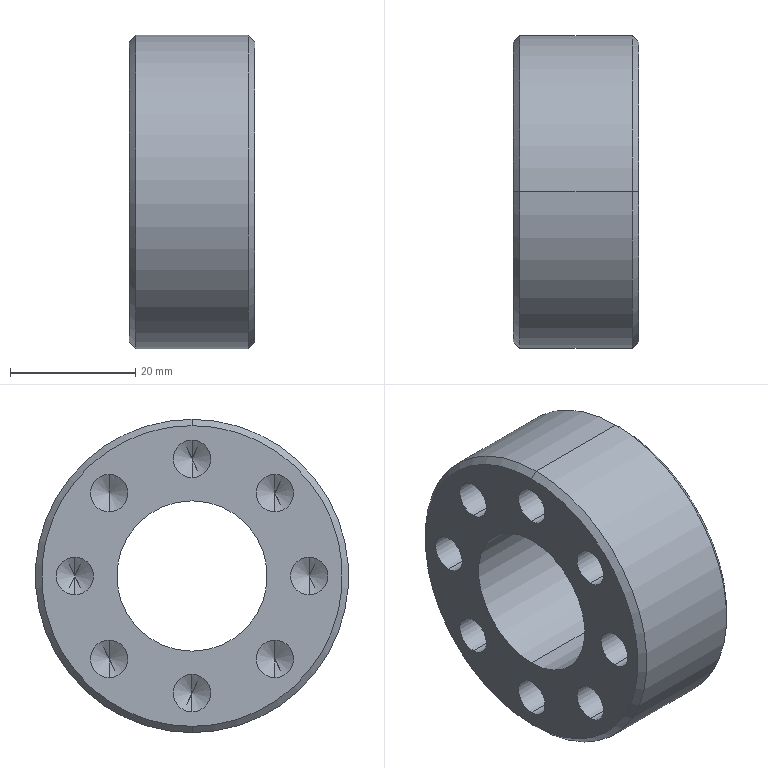Component | SolidWorks | Z24X50X20LockingAssembly-1_Z24X50X20LockingAssembly-1 | 1 solid | 42 faces | box 20 x 50 x 50 mm | volume 26086 mm3 | cone 20 | cylinder 20 | plane 2 | commonest cylinder face diameters 6 x16 24 x2 50 x2
STEP:
#1=CARTESIAN_POINT('',(-1.181,1.378,0.9449));
#2=VERTEX_POINT('',#1);
#3=CARTESIAN_POINT('',(-1.181,1.378,-0.9449));
#4=VERTEX_POINT('',#3);
#5=CARTESIAN_POINT('',(-1.181,1.378,0.));
#6=DIRECTION('',(-1.,-0.,-0.));
#7=DIRECTION('',(0.,0.,1.));
#8=AXIS2_PLACEMENT_3D('',#5,#6,#7);
#9=CIRCLE('',#8,0.9449);
#10=EDGE_CURVE('',#2,#4,#9,.T.);
#11=ORIENTED_EDGE('',*,*,#10,.F.);
#12=CARTESIAN_POINT('',(-1.142,1.378,0.9843));
#13=VERTEX_POINT('',#12);
#14=CARTESIAN_POINT('',(-1.181,1.378,0.9449));
#15=DIRECTION('',(0.7071,0.,0.7071));
#16=VECTOR('',#15,39.37);
#17=LINE('',#14,#16);
#18=EDGE_CURVE('',#2,#13,#17,.T.);
#19=ORIENTED_EDGE('',*,*,#18,.T.);
#20=CARTESIAN_POINT('',(-1.142,1.378,-0.9843));
#21=VERTEX_POINT('',#20);
#22=CARTESIAN_POINT('',(-1.142,1.378,0.));
#23=DIRECTION('',(1.,0.,0.));
#24=DIRECTION('',(0.,0.,1.));
#25=AXIS2_PLACEMENT_3D('',#22,#23,#24);
#26=CIRCLE('',#25,0.9843);
#27=EDGE_CURVE('',#21,#13,#26,.T.);
#28=ORIENTED_EDGE('',*,*,#27,.F.);
#29=CARTESIAN_POINT('',(-1.181,1.378,-0.9449));
#30=DIRECTION('',(0.7071,0.,-0.7071));
#31=VECTOR('',#30,39.37);
#32=LINE('',#29,#31);
#33=EDGE_CURVE('',#4,#21,#32,.T.);
#34=ORIENTED_EDGE('',*,*,#33,.F.);
#35=EDGE_LOOP('',(#11,#19,#28,#34));
#36=FACE_OUTER_BOUND('',#35,.T.);
#37=CARTESIAN_POINT('',(-1.181,1.378,0.));
#38=DIRECTION('',(1.,0.,0.));
#39=DIRECTION('',(0.,0.,-1.));
#40=AXIS2_PLACEMENT_3D('',#37,#38,#39);
#41=CONICAL_SURFACE('',#40,0.9449,0.7854);
#42=ADVANCED_FACE('',(#36),#41,.T.);
#43=CARTESIAN_POINT('',(-0.3937,1.378,-0.9449));
#44=VERTEX_POINT('',#43);
#45=CARTESIAN_POINT('',(-0.3937,1.378,0.9449));
#46=VERTEX_POINT('',#45);
#47=CARTESIAN_POINT('',(-0.3937,1.378,0.));
#48=DIRECTION('',(1.,0.,0.));
#49=DIRECTION('',(0.,0.,1.));
#50=AXIS2_PLACEMENT_3D('',#47,#48,#49);
#51=CIRCLE('',#50,0.9449);
#52=EDGE_CURVE('',#44,#46,#51,.T.);
#53=ORIENTED_EDGE('',*,*,#52,.F.);
#54=CARTESIAN_POINT('',(-0.4331,1.378,-0.9843));
#55=VERTEX_POINT('',#54);
#56=CARTESIAN_POINT('',(-0.4331,1.378,-0.9843));
#57=DIRECTION('',(-0.7071,0.,-0.7071));
#58=VECTOR('',#57,39.37);
#59=LINE('',#56,#58);
#60=EDGE_CURVE('',#44,#55,#59,.T.);
#61=ORIENTED_EDGE('',*,*,#60,.T.);
#62=CARTESIAN_POINT('',(-0.4331,1.378,0.9843));
#63=VERTEX_POINT('',#62);
#64=CARTESIAN_POINT('',(-0.4331,1.378,0.));
#65=DIRECTION('',(-1.,-0.,-0.));
#66=DIRECTION('',(0.,0.,1.));
#67=AXIS2_PLACEMENT_3D('',#64,#65,#66);
#68=CIRCLE('',#67,0.9843);
#69=EDGE_CURVE('',#63,#55,#68,.T.);
#70=ORIENTED_EDGE('',*,*,#69,.F.);
#71=CARTESIAN_POINT('',(-0.4331,1.378,0.9843));
#72=DIRECTION('',(-0.7071,-0.,0.7071));
#73=VECTOR('',#72,39.37);
#74=LINE('',#71,#73);
#75=EDGE_CURVE('',#46,#63,#74,.T.);
#76=ORIENTED_EDGE('',*,*,#75,.F.);
#77=EDGE_LOOP('',(#53,#61,#70,#76));
#78=FACE_OUTER_BOUND('',#77,.T.);
#79=CARTESIAN_POINT('',(-0.4331,1.378,0.));
#80=DIRECTION('',(-1.,-0.,-0.));
#81=DIRECTION('',(0.,0.,1.));
#82=AXIS2_PLACEMENT_3D('',#79,#80,#81);
#83=CONICAL_SURFACE('',#82,0.9843,0.7854);
#84=ADVANCED_FACE('',(#78),#83,.T.);
#85=CARTESIAN_POINT('',(-0.5118,1.378,0.6181));
#86=VERTEX_POINT('',#85);
#87=CARTESIAN_POINT('',(-0.5118,1.378,0.8543));
#88=VERTEX_POINT('',#87);
#89=CARTESIAN_POINT('',(-0.5118,1.378,0.7362));
#90=DIRECTION('',(-1.,-0.,-0.));
#91=DIRECTION('',(0.,0.,1.));
#92=AXIS2_PLACEMENT_3D('',#89,#90,#91);
#93=CIRCLE('',#92,0.1181);
#94=EDGE_CURVE('',#86,#88,#93,.T.);
#95=ORIENTED_EDGE('',*,*,#94,.F.);
#96=CARTESIAN_POINT('',(-1.181,1.378,0.6181));
#97=VERTEX_POINT('',#96);
#98=CARTESIAN_POINT('',(-1.181,1.378,0.6181));
#99=DIRECTION('',(-1.,-0.,-0.));
#100=VECTOR('',#99,39.37);
#101=LINE('',#98,#100);
#102=EDGE_CURVE('',#86,#97,#101,.T.);
#103=ORIENTED_EDGE('',*,*,#102,.T.);
#104=CARTESIAN_POINT('',(-1.181,1.378,0.8543));
#105=VERTEX_POINT('',#104);
#106=CARTESIAN_POINT('',(-1.181,1.378,0.7362));
#107=DIRECTION('',(-1.,-0.,-0.));
#108=DIRECTION('',(0.,0.,1.));
#109=AXIS2_PLACEMENT_3D('',#106,#107,#108);
#110=CIRCLE('',#109,0.1181);
#111=EDGE_CURVE('',#97,#105,#110,.T.);
#112=ORIENTED_EDGE('',*,*,#111,.T.);
#113=CARTESIAN_POINT('',(-1.181,1.378,0.8543));
#114=DIRECTION('',(-1.,-0.,-0.));
#115=VECTOR('',#114,39.37);
#116=LINE('',#113,#115);
#117=EDGE_CURVE('',#88,#105,#116,.T.);
#118=ORIENTED_EDGE('',*,*,#117,.F.);
#119=EDGE_LOOP('',(#95,#103,#112,#118));
#120=FACE_OUTER_BOUND('',#119,.T.);
#121=CARTESIAN_POINT('',(-1.181,1.378,0.7362));
#122=DIRECTION('',(-1.,-0.,-0.));
#123=DIRECTION('',(0.,0.,1.));
#124=AXIS2_PLACEMENT_3D('',#121,#122,#123);
#125=CYLINDRICAL_SURFACE('',#124,0.1181);
#126=ADVANCED_FACE('',(#120),#125,.F.);
#127=CARTESIAN_POINT('',(-0.4408,1.378,0.7362));
#128=VERTEX_POINT('',#127);
#129=CARTESIAN_POINT('',(-0.5118,1.378,0.8543));
#130=DIRECTION('',(-0.515,0.,0.8572));
#131=VECTOR('',#130,39.37);
#132=LINE('',#129,#131);
#133=EDGE_CURVE('',#128,#88,#132,.T.);
#134=ORIENTED_EDGE('',*,*,#133,.F.);
#135=CARTESIAN_POINT('',(-0.5118,1.378,0.6181));
#136=DIRECTION('',(-0.515,0.,-0.8572));
#137=VECTOR('',#136,39.37);
#138=LINE('',#135,#137);
#139=EDGE_CURVE('',#128,#86,#138,.T.);
#140=ORIENTED_EDGE('',*,*,#139,.T.);
#141=ORIENTED_EDGE('',*,*,#94,.T.);
#142=EDGE_LOOP('',(#134,#140,#141));
#143=FACE_OUTER_BOUND('',#142,.T.);
#144=CARTESIAN_POINT('',(-0.5118,1.378,0.7362));
#145=DIRECTION('',(-1.,-0.,-0.));
#146=DIRECTION('',(0.,0.,1.));
#147=AXIS2_PLACEMENT_3D('',#144,#145,#146);
#148=CONICAL_SURFACE('',#147,0.1181,1.03);
#149=ADVANCED_FACE('',(#143),#148,.F.);
#150=CARTESIAN_POINT('',(-0.5118,0.8574,0.4025));
#151=VERTEX_POINT('',#150);
#152=CARTESIAN_POINT('',(-0.5118,0.8574,0.6387));
#153=VERTEX_POINT('',#152);
#154=CARTESIAN_POINT('',(-0.5118,0.8574,0.5206));
#155=DIRECTION('',(-1.,-0.,-0.));
#156=DIRECTION('',(0.,0.,1.));
#157=AXIS2_PLACEMENT_3D('',#154,#155,#156);
#158=CIRCLE('',#157,0.1181);
#159=EDGE_CURVE('',#151,#153,#158,.T.);
#160=ORIENTED_EDGE('',*,*,#159,.F.);
#161=CARTESIAN_POINT('',(-1.181,0.8574,0.4025));
#162=VERTEX_POINT('',#161);
#163=CARTESIAN_POINT('',(-1.181,0.8574,0.4025));
#164=DIRECTION('',(-1.,-0.,-0.));
#165=VECTOR('',#164,39.37);
#166=LINE('',#163,#165);
#167=EDGE_CURVE('',#151,#162,#166,.T.);
#168=ORIENTED_EDGE('',*,*,#167,.T.);
#169=CARTESIAN_POINT('',(-1.181,0.8574,0.6387));
#170=VERTEX_POINT('',#169);
#171=CARTESIAN_POINT('',(-1.181,0.8574,0.5206));
#172=DIRECTION('',(-1.,-0.,-0.));
#173=DIRECTION('',(0.,0.,1.));
#174=AXIS2_PLACEMENT_3D('',#171,#172,#173);
#175=CIRCLE('',#174,0.1181);
#176=EDGE_CURVE('',#162,#170,#175,.T.);
#177=ORIENTED_EDGE('',*,*,#176,.T.);
#178=CARTESIAN_POINT('',(-1.181,0.8574,0.6387));
#179=DIRECTION('',(-1.,-0.,-0.));
#180=VECTOR('',#179,39.37);
#181=LINE('',#178,#180);
#182=EDGE_CURVE('',#153,#170,#181,.T.);
#183=ORIENTED_EDGE('',*,*,#182,.F.);
#184=EDGE_LOOP('',(#160,#168,#177,#183));
#185=FACE_OUTER_BOUND('',#184,.T.);
#186=CARTESIAN_POINT('',(-1.181,0.8574,0.5206));
#187=DIRECTION('',(-1.,-0.,-0.));
#188=DIRECTION('',(0.,0.,1.));
#189=AXIS2_PLACEMENT_3D('',#186,#187,#188);
#190=CYLINDRICAL_SURFACE('',#189,0.1181);
#191=ADVANCED_FACE('',(#185),#190,.F.);
#192=CARTESIAN_POINT('',(-0.4408,0.8574,0.5206));
#193=VERTEX_POINT('',#192);
#194=CARTESIAN_POINT('',(-0.5118,0.8574,0.6387));
#195=DIRECTION('',(-0.515,0.,0.8572));
#196=VECTOR('',#195,39.37);
#197=LINE('',#194,#196);
#198=EDGE_CURVE('',#193,#153,#197,.T.);
#199=ORIENTED_EDGE('',*,*,#198,.F.);
#200=CARTESIAN_POINT('',(-0.5118,0.8574,0.4025));
#201=DIRECTION('',(-0.515,0.,-0.8572));
#202=VECTOR('',#201,39.37);
#203=LINE('',#200,#202);
#204=EDGE_CURVE('',#193,#151,#203,.T.);
#205=ORIENTED_EDGE('',*,*,#204,.T.);
#206=ORIENTED_EDGE('',*,*,#159,.T.);
#207=EDGE_LOOP('',(#199,#205,#206));
#208=FACE_OUTER_BOUND('',#207,.T.);
#209=CARTESIAN_POINT('',(-0.5118,0.8574,0.5206));
#210=DIRECTION('',(-1.,-0.,-0.));
#211=DIRECTION('',(0.,0.,1.));
#212=AXIS2_PLACEMENT_3D('',#209,#210,#211);
#213=CONICAL_SURFACE('',#212,0.1181,1.03);
#214=ADVANCED_FACE('',(#208),#213,.F.);
#215=CARTESIAN_POINT('',(-0.5118,0.6417,-0.1181));
#216=VERTEX_POINT('',#215);
#217=CARTESIAN_POINT('',(-0.5118,0.6417,0.1181));
#218=VERTEX_POINT('',#217);
#219=CARTESIAN_POINT('',(-0.5118,0.6417,-0.));
#220=DIRECTION('',(-1.,-0.,-0.));
#221=DIRECTION('',(0.,0.,1.));
#222=AXIS2_PLACEMENT_3D('',#219,#220,#221);
#223=CIRCLE('',#222,0.1181);
#224=EDGE_CURVE('',#216,#218,#223,.T.);
#225=ORIENTED_EDGE('',*,*,#224,.F.);
#226=CARTESIAN_POINT('',(-1.181,0.6417,-0.1181));
#227=VERTEX_POINT('',#226);
#228=CARTESIAN_POINT('',(-1.181,0.6417,-0.1181));
#229=DIRECTION('',(-1.,-0.,-0.));
#230=VECTOR('',#229,39.37);
#231=LINE('',#228,#230);
#232=EDGE_CURVE('',#216,#227,#231,.T.);
#233=ORIENTED_EDGE('',*,*,#232,.T.);
#234=CARTESIAN_POINT('',(-1.181,0.6417,0.1181));
#235=VERTEX_POINT('',#234);
#236=CARTESIAN_POINT('',(-1.181,0.6417,-0.));
#237=DIRECTION('',(-1.,-0.,-0.));
#238=DIRECTION('',(0.,0.,1.));
#239=AXIS2_PLACEMENT_3D('',#236,#237,#238);
#240=CIRCLE('',#239,0.1181);
#241=EDGE_CURVE('',#227,#235,#240,.T.);
#242=ORIENTED_EDGE('',*,*,#241,.T.);
#243=CARTESIAN_POINT('',(-1.181,0.6417,0.1181));
#244=DIRECTION('',(-1.,-0.,-0.));
#245=VECTOR('',#244,39.37);
#246=LINE('',#243,#245);
#247=EDGE_CURVE('',#218,#235,#246,.T.);
#248=ORIENTED_EDGE('',*,*,#247,.F.);
#249=EDGE_LOOP('',(#225,#233,#242,#248));
#250=FACE_OUTER_BOUND('',#249,.T.);
#251=CARTESIAN_POINT('',(-1.181,0.6417,-0.));
#252=DIRECTION('',(-1.,-0.,-0.));
#253=DIRECTION('',(0.,0.,1.));
#254=AXIS2_PLACEMENT_3D('',#251,#252,#253);
#255=CYLINDRICAL_SURFACE('',#254,0.1181);
#256=ADVANCED_FACE('',(#250),#255,.F.);
#257=CARTESIAN_POINT('',(-0.4408,0.6417,-0.));
#258=VERTEX_POINT('',#257);
#259=CARTESIAN_POINT('',(-0.5118,0.6417,0.1181));
#260=DIRECTION('',(-0.515,0.,0.8572));
#261=VECTOR('',#260,39.37);
#262=LINE('',#259,#261);
#263=EDGE_CURVE('',#258,#218,#262,.T.);
#264=ORIENTED_EDGE('',*,*,#263,.F.);
#265=CARTESIAN_POINT('',(-0.5118,0.6417,-0.1181));
#266=DIRECTION('',(-0.515,0.,-0.8572));
#267=VECTOR('',#266,39.37);
#268=LINE('',#265,#267);
#269=EDGE_CURVE('',#258,#216,#268,.T.);
#270=ORIENTED_EDGE('',*,*,#269,.T.);
#271=ORIENTED_EDGE('',*,*,#224,.T.);
#272=EDGE_LOOP('',(#264,#270,#271));
#273=FACE_OUTER_BOUND('',#272,.T.);
#274=CARTESIAN_POINT('',(-0.5118,0.6417,-0.));
#275=DIRECTION('',(-1.,-0.,-0.));
#276=DIRECTION('',(0.,0.,1.));
#277=AXIS2_PLACEMENT_3D('',#274,#275,#276);
#278=CONICAL_SURFACE('',#277,0.1181,1.03);
#279=ADVANCED_FACE('',(#273),#278,.F.);
#280=CARTESIAN_POINT('',(-0.5118,0.8574,-0.6387));
#281=VERTEX_POINT('',#280);
#282=CARTESIAN_POINT('',(-0.5118,0.8574,-0.4025));
#283=VERTEX_POINT('',#282);
#284=CARTESIAN_POINT('',(-0.5118,0.8574,-0.5206));
#285=DIRECTION('',(-1.,-0.,-0.));
#286=DIRECTION('',(0.,0.,1.));
#287=AXIS2_PLACEMENT_3D('',#284,#285,#286);
#288=CIRCLE('',#287,0.1181);
#289=EDGE_CURVE('',#281,#283,#288,.T.);
#290=ORIENTED_EDGE('',*,*,#289,.F.);
#291=CARTESIAN_POINT('',(-1.181,0.8574,-0.6387));
#292=VERTEX_POINT('',#291);
#293=CARTESIAN_POINT('',(-1.181,0.8574,-0.6387));
#294=DIRECTION('',(-1.,-0.,-0.));
#295=VECTOR('',#294,39.37);
#296=LINE('',#293,#295);
#297=EDGE_CURVE('',#281,#292,#296,.T.);
#298=ORIENTED_EDGE('',*,*,#297,.T.);
#299=CARTESIAN_POINT('',(-1.181,0.8574,-0.4025));
#300=VERTEX_POINT('',#299);
#301=CARTESIAN_POINT('',(-1.181,0.8574,-0.5206));
#302=DIRECTION('',(-1.,-0.,-0.));
#303=DIRECTION('',(0.,0.,1.));
#304=AXIS2_PLACEMENT_3D('',#301,#302,#303);
#305=CIRCLE('',#304,0.1181);
#306=EDGE_CURVE('',#292,#300,#305,.T.);
#307=ORIENTED_EDGE('',*,*,#306,.T.);
#308=CARTESIAN_POINT('',(-1.181,0.8574,-0.4025));
#309=DIRECTION('',(-1.,-0.,-0.));
#310=VECTOR('',#309,39.37);
#311=LINE('',#308,#310);
#312=EDGE_CURVE('',#283,#300,#311,.T.);
#313=ORIENTED_EDGE('',*,*,#312,.F.);
#314=EDGE_LOOP('',(#290,#298,#307,#313));
#315=FACE_OUTER_BOUND('',#314,.T.);
#316=CARTESIAN_POINT('',(-1.181,0.8574,-0.5206));
#317=DIRECTION('',(-1.,-0.,-0.));
#318=DIRECTION('',(0.,0.,1.));
#319=AXIS2_PLACEMENT_3D('',#316,#317,#318);
#320=CYLINDRICAL_SURFACE('',#319,0.1181);
#321=ADVANCED_FACE('',(#315),#320,.F.);
#322=CARTESIAN_POINT('',(-0.4408,0.8574,-0.5206));
#323=VERTEX_POINT('',#322);
#324=CARTESIAN_POINT('',(-0.5118,0.8574,-0.4025));
#325=DIRECTION('',(-0.515,0.,0.8572));
#326=VECTOR('',#325,39.37);
#327=LINE('',#324,#326);
#328=EDGE_CURVE('',#323,#283,#327,.T.);
#329=ORIENTED_EDGE('',*,*,#328,.F.);
#330=CARTESIAN_POINT('',(-0.5118,0.8574,-0.6387));
#331=DIRECTION('',(-0.515,0.,-0.8572));
#332=VECTOR('',#331,39.37);
#333=LINE('',#330,#332);
#334=EDGE_CURVE('',#323,#281,#333,.T.);
#335=ORIENTED_EDGE('',*,*,#334,.T.);
#336=ORIENTED_EDGE('',*,*,#289,.T.);
#337=EDGE_LOOP('',(#329,#335,#336));
#338=FACE_OUTER_BOUND('',#337,.T.);
#339=CARTESIAN_POINT('',(-0.5118,0.8574,-0.5206));
#340=DIRECTION('',(-1.,-0.,-0.));
#341=DIRECTION('',(0.,0.,1.));
#342=AXIS2_PLACEMENT_3D('',#339,#340,#341);
#343=CONICAL_SURFACE('',#342,0.1181,1.03);
#344=ADVANCED_FACE('',(#338),#343,.F.);
#345=CARTESIAN_POINT('',(-0.5118,1.378,-0.8543));
#346=VERTEX_POINT('',#345);
#347=CARTESIAN_POINT('',(-0.5118,1.378,-0.6181));
#348=VERTEX_POINT('',#347);
#349=CARTESIAN_POINT('',(-0.5118,1.378,-0.7362));
#350=DIRECTION('',(-1.,-0.,-0.));
#351=DIRECTION('',(0.,0.,1.));
#352=AXIS2_PLACEMENT_3D('',#349,#350,#351);
#353=CIRCLE('',#352,0.1181);
#354=EDGE_CURVE('',#346,#348,#353,.T.);
#355=ORIENTED_EDGE('',*,*,#354,.F.);
#356=CARTESIAN_POINT('',(-1.181,1.378,-0.8543));
#357=VERTEX_POINT('',#356);
#358=CARTESIAN_POINT('',(-1.181,1.378,-0.8543));
#359=DIRECTION('',(-1.,-0.,-0.));
#360=VECTOR('',#359,39.37);
#361=LINE('',#358,#360);
#362=EDGE_CURVE('',#346,#357,#361,.T.);
#363=ORIENTED_EDGE('',*,*,#362,.T.);
#364=CARTESIAN_POINT('',(-1.181,1.378,-0.6181));
#365=VERTEX_POINT('',#364);
#366=CARTESIAN_POINT('',(-1.181,1.378,-0.7362));
#367=DIRECTION('',(-1.,-0.,-0.));
#368=DIRECTION('',(0.,0.,1.));
#369=AXIS2_PLACEMENT_3D('',#366,#367,#368);
#370=CIRCLE('',#369,0.1181);
#371=EDGE_CURVE('',#357,#365,#370,.T.);
#372=ORIENTED_EDGE('',*,*,#371,.T.);
#373=CARTESIAN_POINT('',(-1.181,1.378,-0.6181));
#374=DIRECTION('',(-1.,-0.,-0.));
#375=VECTOR('',#374,39.37);
#376=LINE('',#373,#375);
#377=EDGE_CURVE('',#348,#365,#376,.T.);
#378=ORIENTED_EDGE('',*,*,#377,.F.);
#379=EDGE_LOOP('',(#355,#363,#372,#378));
#380=FACE_OUTER_BOUND('',#379,.T.);
#381=CARTESIAN_POINT('',(-1.181,1.378,-0.7362));
#382=DIRECTION('',(-1.,-0.,-0.));
#383=DIRECTION('',(0.,0.,1.));
#384=AXIS2_PLACEMENT_3D('',#381,#382,#383);
#385=CYLINDRICAL_SURFACE('',#384,0.1181);
#386=ADVANCED_FACE('',(#380),#385,.F.);
#387=CARTESIAN_POINT('',(-0.4408,1.378,-0.7362));
#388=VERTEX_POINT('',#387);
#389=CARTESIAN_POINT('',(-0.5118,1.378,-0.6181));
#390=DIRECTION('',(-0.515,0.,0.8572));
#391=VECTOR('',#390,39.37);
#392=LINE('',#389,#391);
#393=EDGE_CURVE('',#388,#348,#392,.T.);
#394=ORIENTED_EDGE('',*,*,#393,.F.);
#395=CARTESIAN_POINT('',(-0.5118,1.378,-0.8543));
#396=DIRECTION('',(-0.515,0.,-0.8572));
#397=VECTOR('',#396,39.37);
#398=LINE('',#395,#397);
#399=EDGE_CURVE('',#388,#346,#398,.T.);
#400=ORIENTED_EDGE('',*,*,#399,.T.);
#401=ORIENTED_EDGE('',*,*,#354,.T.);
#402=EDGE_LOOP('',(#394,#400,#401));
#403=FACE_OUTER_BOUND('',#402,.T.);
#404=CARTESIAN_POINT('',(-0.5118,1.378,-0.7362));
#405=DIRECTION('',(-1.,-0.,-0.));
#406=DIRECTION('',(0.,0.,1.));
#407=AXIS2_PLACEMENT_3D('',#404,#405,#406);
#408=CONICAL_SURFACE('',#407,0.1181,1.03);
#409=ADVANCED_FACE('',(#403),#408,.F.);
#410=CARTESIAN_POINT('',(-0.5118,1.899,-0.6387));
#411=VERTEX_POINT('',#410);
#412=CARTESIAN_POINT('',(-0.5118,1.899,-0.4025));
#413=VERTEX_POINT('',#412);
#414=CARTESIAN_POINT('',(-0.5118,1.899,-0.5206));
#415=DIRECTION('',(-1.,-0.,-0.));
#416=DIRECTION('',(0.,0.,1.));
#417=AXIS2_PLACEMENT_3D('',#414,#415,#416);
#418=CIRCLE('',#417,0.1181);
#419=EDGE_CURVE('',#411,#413,#418,.T.);
#420=ORIENTED_EDGE('',*,*,#419,.F.);
#421=CARTESIAN_POINT('',(-1.181,1.899,-0.6387));
#422=VERTEX_POINT('',#421);
#423=CARTESIAN_POINT('',(-1.181,1.899,-0.6387));
#424=DIRECTION('',(-1.,-0.,-0.));
#425=VECTOR('',#424,39.37);
#426=LINE('',#423,#425);
#427=EDGE_CURVE('',#411,#422,#426,.T.);
#428=ORIENTED_EDGE('',*,*,#427,.T.);
#429=CARTESIAN_POINT('',(-1.181,1.899,-0.4025));
#430=VERTEX_POINT('',#429);
#431=CARTESIAN_POINT('',(-1.181,1.899,-0.5206));
#432=DIRECTION('',(-1.,-0.,-0.));
#433=DIRECTION('',(0.,0.,1.));
#434=AXIS2_PLACEMENT_3D('',#431,#432,#433);
#435=CIRCLE('',#434,0.1181);
#436=EDGE_CURVE('',#422,#430,#435,.T.);
#437=ORIENTED_EDGE('',*,*,#436,.T.);
#438=CARTESIAN_POINT('',(-1.181,1.899,-0.4025));
#439=DIRECTION('',(-1.,-0.,-0.));
#440=VECTOR('',#439,39.37);
#441=LINE('',#438,#440);
#442=EDGE_CURVE('',#413,#430,#441,.T.);
#443=ORIENTED_EDGE('',*,*,#442,.F.);
#444=EDGE_LOOP('',(#420,#428,#437,#443));
#445=FACE_OUTER_BOUND('',#444,.T.);
#446=CARTESIAN_POINT('',(-1.181,1.899,-0.5206));
#447=DIRECTION('',(-1.,-0.,-0.));
#448=DIRECTION('',(0.,0.,1.));
#449=AXIS2_PLACEMENT_3D('',#446,#447,#448);
#450=CYLINDRICAL_SURFACE('',#449,0.1181);
#451=ADVANCED_FACE('',(#445),#450,.F.);
#452=CARTESIAN_POINT('',(-0.4408,1.899,-0.5206));
#453=VERTEX_POINT('',#452);
#454=CARTESIAN_POINT('',(-0.5118,1.899,-0.4025));
#455=DIRECTION('',(-0.515,0.,0.8572));
#456=VECTOR('',#455,39.37);
#457=LINE('',#454,#456);
#458=EDGE_CURVE('',#453,#413,#457,.T.);
#459=ORIENTED_EDGE('',*,*,#458,.F.);
#460=CARTESIAN_POINT('',(-0.5118,1.899,-0.6387));
#461=DIRECTION('',(-0.515,0.,-0.8572));
#462=VECTOR('',#461,39.37);
#463=LINE('',#460,#462);
#464=EDGE_CURVE('',#453,#411,#463,.T.);
#465=ORIENTED_EDGE('',*,*,#464,.T.);
#466=ORIENTED_EDGE('',*,*,#419,.T.);
#467=EDGE_LOOP('',(#459,#465,#466));
#468=FACE_OUTER_BOUND('',#467,.T.);
#469=CARTESIAN_POINT('',(-0.5118,1.899,-0.5206));
#470=DIRECTION('',(-1.,-0.,-0.));
#471=DIRECTION('',(0.,0.,1.));
#472=AXIS2_PLACEMENT_3D('',#469,#470,#471);
#473=CONICAL_SURFACE('',#472,0.1181,1.03);
#474=ADVANCED_FACE('',(#468),#473,.F.);
#475=CARTESIAN_POINT('',(-0.5118,2.114,-0.1181));
#476=VERTEX_POINT('',#475);
#477=CARTESIAN_POINT('',(-0.5118,2.114,0.1181));
#478=VERTEX_POINT('',#477);
#479=CARTESIAN_POINT('',(-0.5118,2.114,0.));
#480=DIRECTION('',(-1.,-0.,-0.));
#481=DIRECTION('',(0.,0.,1.));
#482=AXIS2_PLACEMENT_3D('',#479,#480,#481);
#483=CIRCLE('',#482,0.1181);
#484=EDGE_CURVE('',#476,#478,#483,.T.);
#485=ORIENTED_EDGE('',*,*,#484,.F.);
#486=CARTESIAN_POINT('',(-1.181,2.114,-0.1181));
#487=VERTEX_POINT('',#486);
#488=CARTESIAN_POINT('',(-1.181,2.114,-0.1181));
#489=DIRECTION('',(-1.,-0.,-0.));
#490=VECTOR('',#489,39.37);
#491=LINE('',#488,#490);
#492=EDGE_CURVE('',#476,#487,#491,.T.);
#493=ORIENTED_EDGE('',*,*,#492,.T.);
#494=CARTESIAN_POINT('',(-1.181,2.114,0.1181));
#495=VERTEX_POINT('',#494);
#496=CARTESIAN_POINT('',(-1.181,2.114,0.));
#497=DIRECTION('',(-1.,-0.,-0.));
#498=DIRECTION('',(0.,0.,1.));
#499=AXIS2_PLACEMENT_3D('',#496,#497,#498);
#500=CIRCLE('',#499,0.1181);
#501=EDGE_CURVE('',#487,#495,#500,.T.);
#502=ORIENTED_EDGE('',*,*,#501,.T.);
#503=CARTESIAN_POINT('',(-1.181,2.114,0.1181));
#504=DIRECTION('',(-1.,-0.,-0.));
#505=VECTOR('',#504,39.37);
#506=LINE('',#503,#505);
#507=EDGE_CURVE('',#478,#495,#506,.T.);
#508=ORIENTED_EDGE('',*,*,#507,.F.);
#509=EDGE_LOOP('',(#485,#493,#502,#508));
#510=FACE_OUTER_BOUND('',#509,.T.);
#511=CARTESIAN_POINT('',(-1.181,2.114,0.));
#512=DIRECTION('',(-1.,-0.,-0.));
#513=DIRECTION('',(0.,0.,1.));
#514=AXIS2_PLACEMENT_3D('',#511,#512,#513);
#515=CYLINDRICAL_SURFACE('',#514,0.1181);
#516=ADVANCED_FACE('',(#510),#515,.F.);
#517=CARTESIAN_POINT('',(-0.4408,2.114,0.));
#518=VERTEX_POINT('',#517);
#519=CARTESIAN_POINT('',(-0.5118,2.114,0.1181));
#520=DIRECTION('',(-0.515,0.,0.8572));
#521=VECTOR('',#520,39.37);
#522=LINE('',#519,#521);
#523=EDGE_CURVE('',#518,#478,#522,.T.);
#524=ORIENTED_EDGE('',*,*,#523,.F.);
#525=CARTESIAN_POINT('',(-0.5118,2.114,-0.1181));
#526=DIRECTION('',(-0.515,0.,-0.8572));
#527=VECTOR('',#526,39.37);
#528=LINE('',#525,#527);
#529=EDGE_CURVE('',#518,#476,#528,.T.);
#530=ORIENTED_EDGE('',*,*,#529,.T.);
#531=ORIENTED_EDGE('',*,*,#484,.T.);
#532=EDGE_LOOP('',(#524,#530,#531));
#533=FACE_OUTER_BOUND('',#532,.T.);
#534=CARTESIAN_POINT('',(-0.5118,2.114,0.));
#535=DIRECTION('',(-1.,-0.,-0.));
#536=DIRECTION('',(0.,0.,1.));
#537=AXIS2_PLACEMENT_3D('',#534,#535,#536);
#538=CONICAL_SURFACE('',#537,0.1181,1.03);
#539=ADVANCED_FACE('',(#533),#538,.F.);
#540=CARTESIAN_POINT('',(-0.5118,1.899,0.4025));
#541=VERTEX_POINT('',#540);
#542=CARTESIAN_POINT('',(-0.5118,1.899,0.6387));
#543=VERTEX_POINT('',#542);
#544=CARTESIAN_POINT('',(-0.5118,1.899,0.5206));
#545=DIRECTION('',(-1.,-0.,-0.));
#546=DIRECTION('',(0.,0.,1.));
#547=AXIS2_PLACEMENT_3D('',#544,#545,#546);
#548=CIRCLE('',#547,0.1181);
#549=EDGE_CURVE('',#541,#543,#548,.T.);
#550=ORIENTED_EDGE('',*,*,#549,.F.);
#551=CARTESIAN_POINT('',(-1.181,1.899,0.4025));
#552=VERTEX_POINT('',#551);
#553=CARTESIAN_POINT('',(-1.181,1.899,0.4025));
#554=DIRECTION('',(-1.,-0.,-0.));
#555=VECTOR('',#554,39.37);
#556=LINE('',#553,#555);
#557=EDGE_CURVE('',#541,#552,#556,.T.);
#558=ORIENTED_EDGE('',*,*,#557,.T.);
#559=CARTESIAN_POINT('',(-1.181,1.899,0.6387));
#560=VERTEX_POINT('',#559);
#561=CARTESIAN_POINT('',(-1.181,1.899,0.5206));
#562=DIRECTION('',(-1.,-0.,-0.));
#563=DIRECTION('',(0.,0.,1.));
#564=AXIS2_PLACEMENT_3D('',#561,#562,#563);
#565=CIRCLE('',#564,0.1181);
#566=EDGE_CURVE('',#552,#560,#565,.T.);
#567=ORIENTED_EDGE('',*,*,#566,.T.);
#568=CARTESIAN_POINT('',(-1.181,1.899,0.6387));
#569=DIRECTION('',(-1.,-0.,-0.));
#570=VECTOR('',#569,39.37);
#571=LINE('',#568,#570);
#572=EDGE_CURVE('',#543,#560,#571,.T.);
#573=ORIENTED_EDGE('',*,*,#572,.F.);
#574=EDGE_LOOP('',(#550,#558,#567,#573));
#575=FACE_OUTER_BOUND('',#574,.T.);
#576=CARTESIAN_POINT('',(-1.181,1.899,0.5206));
#577=DIRECTION('',(-1.,-0.,-0.));
#578=DIRECTION('',(0.,0.,1.));
#579=AXIS2_PLACEMENT_3D('',#576,#577,#578);
#580=CYLINDRICAL_SURFACE('',#579,0.1181);
#581=ADVANCED_FACE('',(#575),#580,.F.);
#582=CARTESIAN_POINT('',(-0.4408,1.899,0.5206));
#583=VERTEX_POINT('',#582);
#584=CARTESIAN_POINT('',(-0.5118,1.899,0.6387));
#585=DIRECTION('',(-0.515,0.,0.8572));
#586=VECTOR('',#585,39.37);
#587=LINE('',#584,#586);
#588=EDGE_CURVE('',#583,#543,#587,.T.);
#589=ORIENTED_EDGE('',*,*,#588,.F.);
#590=CARTESIAN_POINT('',(-0.5118,1.899,0.4025));
#591=DIRECTION('',(-0.515,0.,-0.8572));
#592=VECTOR('',#591,39.37);
#593=LINE('',#590,#592);
#594=EDGE_CURVE('',#583,#541,#593,.T.);
#595=ORIENTED_EDGE('',*,*,#594,.T.);
#596=ORIENTED_EDGE('',*,*,#549,.T.);
#597=EDGE_LOOP('',(#589,#595,#596));
#598=FACE_OUTER_BOUND('',#597,.T.);
#599=CARTESIAN_POINT('',(-0.5118,1.899,0.5206));
#600=DIRECTION('',(-1.,-0.,-0.));
#601=DIRECTION('',(0.,0.,1.));
#602=AXIS2_PLACEMENT_3D('',#599,#600,#601);
#603=CONICAL_SURFACE('',#602,0.1181,1.03);
#604=ADVANCED_FACE('',(#598),#603,.F.);
#605=CARTESIAN_POINT('',(-1.181,1.378,-0.4724));
#606=VERTEX_POINT('',#605);
#607=CARTESIAN_POINT('',(-1.181,1.378,0.4724));
#608=VERTEX_POINT('',#607);
#609=CARTESIAN_POINT('',(-1.181,1.378,0.));
#610=DIRECTION('',(-1.,-0.,-0.));
#611=DIRECTION('',(0.,0.,1.));
#612=AXIS2_PLACEMENT_3D('',#609,#610,#611);
#613=CIRCLE('',#612,0.4724);
#614=EDGE_CURVE('',#606,#608,#613,.T.);
#615=ORIENTED_EDGE('',*,*,#614,.T.);
#616=CARTESIAN_POINT('',(-0.3937,1.378,0.4724));
#617=VERTEX_POINT('',#616);
#618=CARTESIAN_POINT('',(-1.181,1.378,0.4724));
#619=DIRECTION('',(1.,0.,0.));
#620=VECTOR('',#619,39.37);
#621=LINE('',#618,#620);
#622=EDGE_CURVE('',#608,#617,#621,.T.);
#623=ORIENTED_EDGE('',*,*,#622,.T.);
#624=CARTESIAN_POINT('',(-0.3937,1.378,-0.4724));
#625=VERTEX_POINT('',#624);
#626=CARTESIAN_POINT('',(-0.3937,1.378,0.));
#627=DIRECTION('',(-1.,-0.,-0.));
#628=DIRECTION('',(0.,0.,1.));
#629=AXIS2_PLACEMENT_3D('',#626,#627,#628);
#630=CIRCLE('',#629,0.4724);
#631=EDGE_CURVE('',#625,#617,#630,.T.);
#632=ORIENTED_EDGE('',*,*,#631,.F.);
#633=CARTESIAN_POINT('',(-1.181,1.378,-0.4724));
#634=DIRECTION('',(1.,0.,0.));
#635=VECTOR('',#634,39.37);
#636=LINE('',#633,#635);
#637=EDGE_CURVE('',#606,#625,#636,.T.);
#638=ORIENTED_EDGE('',*,*,#637,.F.);
#639=EDGE_LOOP('',(#615,#623,#632,#638));
#640=FACE_OUTER_BOUND('',#639,.T.);
#641=CARTESIAN_POINT('',(-1.181,1.378,0.));
#642=DIRECTION('',(1.,0.,0.));
#643=DIRECTION('',(0.,0.,-1.));
#644=AXIS2_PLACEMENT_3D('',#641,#642,#643);
#645=CYLINDRICAL_SURFACE('',#644,0.4724);
#646=ADVANCED_FACE('',(#640),#645,.F.);
#647=ORIENTED_EDGE('',*,*,#27,.T.);
#648=CARTESIAN_POINT('',(-1.181,1.378,0.9843));
#649=DIRECTION('',(1.,0.,0.));
#650=VECTOR('',#649,39.37);
#651=LINE('',#648,#650);
#652=EDGE_CURVE('',#13,#63,#651,.T.);
#653=ORIENTED_EDGE('',*,*,#652,.T.);
#654=ORIENTED_EDGE('',*,*,#69,.T.);
#655=CARTESIAN_POINT('',(-1.181,1.378,-0.9843));
#656=DIRECTION('',(1.,0.,0.));
#657=VECTOR('',#656,39.37);
#658=LINE('',#655,#657);
#659=EDGE_CURVE('',#21,#55,#658,.T.);
#660=ORIENTED_EDGE('',*,*,#659,.F.);
#661=EDGE_LOOP('',(#647,#653,#654,#660));
#662=FACE_OUTER_BOUND('',#661,.T.);
#663=CARTESIAN_POINT('',(-1.181,1.378,0.));
#664=DIRECTION('',(1.,0.,0.));
#665=DIRECTION('',(0.,0.,-1.));
#666=AXIS2_PLACEMENT_3D('',#663,#664,#665);
#667=CYLINDRICAL_SURFACE('',#666,0.9843);
#668=ADVANCED_FACE('',(#662),#667,.T.);
#669=CARTESIAN_POINT('',(-1.181,1.378,0.));
#670=DIRECTION('',(-1.,-0.,-0.));
#671=DIRECTION('',(0.,0.,1.));
#672=AXIS2_PLACEMENT_3D('',#669,#670,#671);
#673=CIRCLE('',#672,0.9449);
#674=EDGE_CURVE('',#4,#2,#673,.T.);
#675=ORIENTED_EDGE('',*,*,#674,.T.);
#676=ORIENTED_EDGE('',*,*,#10,.T.);
#677=EDGE_LOOP('',(#675,#676));
#678=FACE_OUTER_BOUND('',#677,.T.);
#679=CARTESIAN_POINT('',(-1.181,1.378,0.7362));
#680=DIRECTION('',(-1.,-0.,-0.));
#681=DIRECTION('',(0.,0.,1.));
#682=AXIS2_PLACEMENT_3D('',#679,#680,#681);
#683=CIRCLE('',#682,0.1181);
#684=EDGE_CURVE('',#105,#97,#683,.T.);
#685=ORIENTED_EDGE('',*,*,#684,.F.);
#686=ORIENTED_EDGE('',*,*,#111,.F.);
#687=EDGE_LOOP('',(#685,#686));
#688=FACE_BOUND('',#687,.T.);
#689=CARTESIAN_POINT('',(-1.181,0.8574,0.5206));
#690=DIRECTION('',(-1.,-0.,-0.));
#691=DIRECTION('',(0.,0.,1.));
#692=AXIS2_PLACEMENT_3D('',#689,#690,#691);
#693=CIRCLE('',#692,0.1181);
#694=EDGE_CURVE('',#170,#162,#693,.T.);
#695=ORIENTED_EDGE('',*,*,#694,.F.);
#696=ORIENTED_EDGE('',*,*,#176,.F.);
#697=EDGE_LOOP('',(#695,#696));
#698=FACE_BOUND('',#697,.T.);
#699=CARTESIAN_POINT('',(-1.181,0.6417,-0.));
#700=DIRECTION('',(-1.,-0.,-0.));
#701=DIRECTION('',(0.,0.,1.));
#702=AXIS2_PLACEMENT_3D('',#699,#700,#701);
#703=CIRCLE('',#702,0.1181);
#704=EDGE_CURVE('',#235,#227,#703,.T.);
#705=ORIENTED_EDGE('',*,*,#704,.F.);
#706=ORIENTED_EDGE('',*,*,#241,.F.);
#707=EDGE_LOOP('',(#705,#706));
#708=FACE_BOUND('',#707,.T.);
#709=CARTESIAN_POINT('',(-1.181,0.8574,-0.5206));
#710=DIRECTION('',(-1.,-0.,-0.));
#711=DIRECTION('',(0.,0.,1.));
#712=AXIS2_PLACEMENT_3D('',#709,#710,#711);
#713=CIRCLE('',#712,0.1181);
#714=EDGE_CURVE('',#300,#292,#713,.T.);
#715=ORIENTED_EDGE('',*,*,#714,.F.);
#716=ORIENTED_EDGE('',*,*,#306,.F.);
#717=EDGE_LOOP('',(#715,#716));
#718=FACE_BOUND('',#717,.T.);
#719=CARTESIAN_POINT('',(-1.181,1.378,-0.7362));
#720=DIRECTION('',(-1.,-0.,-0.));
#721=DIRECTION('',(0.,0.,1.));
#722=AXIS2_PLACEMENT_3D('',#719,#720,#721);
#723=CIRCLE('',#722,0.1181);
#724=EDGE_CURVE('',#365,#357,#723,.T.);
#725=ORIENTED_EDGE('',*,*,#724,.F.);
#726=ORIENTED_EDGE('',*,*,#371,.F.);
#727=EDGE_LOOP('',(#725,#726));
#728=FACE_BOUND('',#727,.T.);
#729=CARTESIAN_POINT('',(-1.181,1.899,-0.5206));
#730=DIRECTION('',(-1.,-0.,-0.));
#731=DIRECTION('',(0.,0.,1.));
#732=AXIS2_PLACEMENT_3D('',#729,#730,#731);
#733=CIRCLE('',#732,0.1181);
#734=EDGE_CURVE('',#430,#422,#733,.T.);
#735=ORIENTED_EDGE('',*,*,#734,.F.);
#736=ORIENTED_EDGE('',*,*,#436,.F.);
#737=EDGE_LOOP('',(#735,#736));
#738=FACE_BOUND('',#737,.T.);
#739=CARTESIAN_POINT('',(-1.181,2.114,0.));
#740=DIRECTION('',(-1.,-0.,-0.));
#741=DIRECTION('',(0.,0.,1.));
#742=AXIS2_PLACEMENT_3D('',#739,#740,#741);
#743=CIRCLE('',#742,0.1181);
#744=EDGE_CURVE('',#495,#487,#743,.T.);
#745=ORIENTED_EDGE('',*,*,#744,.F.);
#746=ORIENTED_EDGE('',*,*,#501,.F.);
#747=EDGE_LOOP('',(#745,#746));
#748=FACE_BOUND('',#747,.T.);
#749=CARTESIAN_POINT('',(-1.181,1.899,0.5206));
#750=DIRECTION('',(-1.,-0.,-0.));
#751=DIRECTION('',(0.,0.,1.));
#752=AXIS2_PLACEMENT_3D('',#749,#750,#751);
#753=CIRCLE('',#752,0.1181);
#754=EDGE_CURVE('',#560,#552,#753,.T.);
#755=ORIENTED_EDGE('',*,*,#754,.F.);
#756=ORIENTED_EDGE('',*,*,#566,.F.);
#757=EDGE_LOOP('',(#755,#756));
#758=FACE_BOUND('',#757,.T.);
#759=ORIENTED_EDGE('',*,*,#614,.F.);
#760=CARTESIAN_POINT('',(-1.181,1.378,0.));
#761=DIRECTION('',(-1.,-0.,-0.));
#762=DIRECTION('',(0.,0.,1.));
#763=AXIS2_PLACEMENT_3D('',#760,#761,#762);
#764=CIRCLE('',#763,0.4724);
#765=EDGE_CURVE('',#608,#606,#764,.T.);
#766=ORIENTED_EDGE('',*,*,#765,.F.);
#767=EDGE_LOOP('',(#759,#766));
#768=FACE_BOUND('',#767,.T.);
#769=CARTESIAN_POINT('',(-1.181,1.378,0.));
#770=DIRECTION('',(-1.,-0.,-0.));
#771=DIRECTION('',(-0.,0.,1.));
#772=AXIS2_PLACEMENT_3D('',#769,#770,#771);
#773=PLANE('',#772);
#774=ADVANCED_FACE('',(#678,#688,#698,#708,#718,#728,#738,#748,#758,#768),#773,.T.);
#775=CARTESIAN_POINT('',(-0.3937,1.378,0.));
#776=DIRECTION('',(1.,0.,0.));
#777=DIRECTION('',(0.,0.,1.));
#778=AXIS2_PLACEMENT_3D('',#775,#776,#777);
#779=CIRCLE('',#778,0.9449);
#780=EDGE_CURVE('',#46,#44,#779,.T.);
#781=ORIENTED_EDGE('',*,*,#780,.T.);
#782=ORIENTED_EDGE('',*,*,#52,.T.);
#783=EDGE_LOOP('',(#781,#782));
#784=FACE_OUTER_BOUND('',#783,.T.);
#785=ORIENTED_EDGE('',*,*,#631,.T.);
#786=CARTESIAN_POINT('',(-0.3937,1.378,0.));
#787=DIRECTION('',(-1.,-0.,-0.));
#788=DIRECTION('',(0.,0.,1.));
#789=AXIS2_PLACEMENT_3D('',#786,#787,#788);
#790=CIRCLE('',#789,0.4724);
#791=EDGE_CURVE('',#617,#625,#790,.T.);
#792=ORIENTED_EDGE('',*,*,#791,.T.);
#793=EDGE_LOOP('',(#785,#792));
#794=FACE_BOUND('',#793,.T.);
#795=CARTESIAN_POINT('',(-0.3937,1.378,0.));
#796=DIRECTION('',(-1.,-0.,-0.));
#797=DIRECTION('',(-0.,0.,1.));
#798=AXIS2_PLACEMENT_3D('',#795,#796,#797);
#799=PLANE('',#798);
#800=ADVANCED_FACE('',(#784,#794),#799,.F.);
#801=ORIENTED_EDGE('',*,*,#652,.F.);
#802=CARTESIAN_POINT('',(-1.142,1.378,0.));
#803=DIRECTION('',(1.,0.,0.));
#804=DIRECTION('',(0.,0.,1.));
#805=AXIS2_PLACEMENT_3D('',#802,#803,#804);
#806=CIRCLE('',#805,0.9843);
#807=EDGE_CURVE('',#13,#21,#806,.T.);
#808=ORIENTED_EDGE('',*,*,#807,.T.);
#809=ORIENTED_EDGE('',*,*,#659,.T.);
#810=CARTESIAN_POINT('',(-0.4331,1.378,0.));
#811=DIRECTION('',(-1.,-0.,-0.));
#812=DIRECTION('',(0.,0.,1.));
#813=AXIS2_PLACEMENT_3D('',#810,#811,#812);
#814=CIRCLE('',#813,0.9843);
#815=EDGE_CURVE('',#55,#63,#814,.T.);
#816=ORIENTED_EDGE('',*,*,#815,.T.);
#817=EDGE_LOOP('',(#801,#808,#809,#816));
#818=FACE_OUTER_BOUND('',#817,.T.);
#819=CARTESIAN_POINT('',(-1.181,1.378,0.));
#820=DIRECTION('',(1.,0.,0.));
#821=DIRECTION('',(0.,0.,-1.));
#822=AXIS2_PLACEMENT_3D('',#819,#820,#821);
#823=CYLINDRICAL_SURFACE('',#822,0.9843);
#824=ADVANCED_FACE('',(#818),#823,.T.);
#825=ORIENTED_EDGE('',*,*,#622,.F.);
#826=ORIENTED_EDGE('',*,*,#765,.T.);
#827=ORIENTED_EDGE('',*,*,#637,.T.);
#828=ORIENTED_EDGE('',*,*,#791,.F.);
#829=EDGE_LOOP('',(#825,#826,#827,#828));
#830=FACE_OUTER_BOUND('',#829,.T.);
#831=CARTESIAN_POINT('',(-1.181,1.378,0.));
#832=DIRECTION('',(1.,0.,0.));
#833=DIRECTION('',(0.,0.,-1.));
#834=AXIS2_PLACEMENT_3D('',#831,#832,#833);
#835=CYLINDRICAL_SURFACE('',#834,0.4724);
#836=ADVANCED_FACE('',(#830),#835,.F.);
#837=ORIENTED_EDGE('',*,*,#594,.F.);
#838=ORIENTED_EDGE('',*,*,#588,.T.);
#839=CARTESIAN_POINT('',(-0.5118,1.899,0.5206));
#840=DIRECTION('',(-1.,-0.,-0.));
#841=DIRECTION('',(0.,0.,1.));
#842=AXIS2_PLACEMENT_3D('',#839,#840,#841);
#843=CIRCLE('',#842,0.1181);
#844=EDGE_CURVE('',#543,#541,#843,.T.);
#845=ORIENTED_EDGE('',*,*,#844,.T.);
#846=EDGE_LOOP('',(#837,#838,#845));
#847=FACE_OUTER_BOUND('',#846,.T.);
#848=CARTESIAN_POINT('',(-0.5118,1.899,0.5206));
#849=DIRECTION('',(-1.,-0.,-0.));
#850=DIRECTION('',(0.,0.,1.));
#851=AXIS2_PLACEMENT_3D('',#848,#849,#850);
#852=CONICAL_SURFACE('',#851,0.1181,1.03);
#853=ADVANCED_FACE('',(#847),#852,.F.);
#854=ORIENTED_EDGE('',*,*,#557,.F.);
#855=ORIENTED_EDGE('',*,*,#844,.F.);
#856=ORIENTED_EDGE('',*,*,#572,.T.);
#857=ORIENTED_EDGE('',*,*,#754,.T.);
#858=EDGE_LOOP('',(#854,#855,#856,#857));
#859=FACE_OUTER_BOUND('',#858,.T.);
#860=CARTESIAN_POINT('',(-1.181,1.899,0.5206));
#861=DIRECTION('',(-1.,-0.,-0.));
#862=DIRECTION('',(0.,0.,1.));
#863=AXIS2_PLACEMENT_3D('',#860,#861,#862);
#864=CYLINDRICAL_SURFACE('',#863,0.1181);
#865=ADVANCED_FACE('',(#859),#864,.F.);
#866=ORIENTED_EDGE('',*,*,#529,.F.);
#867=ORIENTED_EDGE('',*,*,#523,.T.);
#868=CARTESIAN_POINT('',(-0.5118,2.114,0.));
#869=DIRECTION('',(-1.,-0.,-0.));
#870=DIRECTION('',(0.,0.,1.));
#871=AXIS2_PLACEMENT_3D('',#868,#869,#870);
#872=CIRCLE('',#871,0.1181);
#873=EDGE_CURVE('',#478,#476,#872,.T.);
#874=ORIENTED_EDGE('',*,*,#873,.T.);
#875=EDGE_LOOP('',(#866,#867,#874));
#876=FACE_OUTER_BOUND('',#875,.T.);
#877=CARTESIAN_POINT('',(-0.5118,2.114,0.));
#878=DIRECTION('',(-1.,-0.,-0.));
#879=DIRECTION('',(0.,0.,1.));
#880=AXIS2_PLACEMENT_3D('',#877,#878,#879);
#881=CONICAL_SURFACE('',#880,0.1181,1.03);
#882=ADVANCED_FACE('',(#876),#881,.F.);
#883=ORIENTED_EDGE('',*,*,#492,.F.);
#884=ORIENTED_EDGE('',*,*,#873,.F.);
#885=ORIENTED_EDGE('',*,*,#507,.T.);
#886=ORIENTED_EDGE('',*,*,#744,.T.);
#887=EDGE_LOOP('',(#883,#884,#885,#886));
#888=FACE_OUTER_BOUND('',#887,.T.);
#889=CARTESIAN_POINT('',(-1.181,2.114,0.));
#890=DIRECTION('',(-1.,-0.,-0.));
#891=DIRECTION('',(0.,0.,1.));
#892=AXIS2_PLACEMENT_3D('',#889,#890,#891);
#893=CYLINDRICAL_SURFACE('',#892,0.1181);
#894=ADVANCED_FACE('',(#888),#893,.F.);
#895=ORIENTED_EDGE('',*,*,#464,.F.);
#896=ORIENTED_EDGE('',*,*,#458,.T.);
#897=CARTESIAN_POINT('',(-0.5118,1.899,-0.5206));
#898=DIRECTION('',(-1.,-0.,-0.));
#899=DIRECTION('',(0.,0.,1.));
#900=AXIS2_PLACEMENT_3D('',#897,#898,#899);
#901=CIRCLE('',#900,0.1181);
#902=EDGE_CURVE('',#413,#411,#901,.T.);
#903=ORIENTED_EDGE('',*,*,#902,.T.);
#904=EDGE_LOOP('',(#895,#896,#903));
#905=FACE_OUTER_BOUND('',#904,.T.);
#906=CARTESIAN_POINT('',(-0.5118,1.899,-0.5206));
#907=DIRECTION('',(-1.,-0.,-0.));
#908=DIRECTION('',(0.,0.,1.));
#909=AXIS2_PLACEMENT_3D('',#906,#907,#908);
#910=CONICAL_SURFACE('',#909,0.1181,1.03);
#911=ADVANCED_FACE('',(#905),#910,.F.);
#912=ORIENTED_EDGE('',*,*,#427,.F.);
#913=ORIENTED_EDGE('',*,*,#902,.F.);
#914=ORIENTED_EDGE('',*,*,#442,.T.);
#915=ORIENTED_EDGE('',*,*,#734,.T.);
#916=EDGE_LOOP('',(#912,#913,#914,#915));
#917=FACE_OUTER_BOUND('',#916,.T.);
#918=CARTESIAN_POINT('',(-1.181,1.899,-0.5206));
#919=DIRECTION('',(-1.,-0.,-0.));
#920=DIRECTION('',(0.,0.,1.));
#921=AXIS2_PLACEMENT_3D('',#918,#919,#920);
#922=CYLINDRICAL_SURFACE('',#921,0.1181);
#923=ADVANCED_FACE('',(#917),#922,.F.);
#924=ORIENTED_EDGE('',*,*,#399,.F.);
#925=ORIENTED_EDGE('',*,*,#393,.T.);
#926=CARTESIAN_POINT('',(-0.5118,1.378,-0.7362));
#927=DIRECTION('',(-1.,-0.,-0.));
#928=DIRECTION('',(0.,0.,1.));
#929=AXIS2_PLACEMENT_3D('',#926,#927,#928);
#930=CIRCLE('',#929,0.1181);
#931=EDGE_CURVE('',#348,#346,#930,.T.);
#932=ORIENTED_EDGE('',*,*,#931,.T.);
#933=EDGE_LOOP('',(#924,#925,#932));
#934=FACE_OUTER_BOUND('',#933,.T.);
#935=CARTESIAN_POINT('',(-0.5118,1.378,-0.7362));
#936=DIRECTION('',(-1.,-0.,-0.));
#937=DIRECTION('',(0.,0.,1.));
#938=AXIS2_PLACEMENT_3D('',#935,#936,#937);
#939=CONICAL_SURFACE('',#938,0.1181,1.03);
#940=ADVANCED_FACE('',(#934),#939,.F.);
#941=ORIENTED_EDGE('',*,*,#362,.F.);
#942=ORIENTED_EDGE('',*,*,#931,.F.);
#943=ORIENTED_EDGE('',*,*,#377,.T.);
#944=ORIENTED_EDGE('',*,*,#724,.T.);
#945=EDGE_LOOP('',(#941,#942,#943,#944));
#946=FACE_OUTER_BOUND('',#945,.T.);
#947=CARTESIAN_POINT('',(-1.181,1.378,-0.7362));
#948=DIRECTION('',(-1.,-0.,-0.));
#949=DIRECTION('',(0.,0.,1.));
#950=AXIS2_PLACEMENT_3D('',#947,#948,#949);
#951=CYLINDRICAL_SURFACE('',#950,0.1181);
#952=ADVANCED_FACE('',(#946),#951,.F.);
#953=ORIENTED_EDGE('',*,*,#334,.F.);
#954=ORIENTED_EDGE('',*,*,#328,.T.);
#955=CARTESIAN_POINT('',(-0.5118,0.8574,-0.5206));
#956=DIRECTION('',(-1.,-0.,-0.));
#957=DIRECTION('',(0.,0.,1.));
#958=AXIS2_PLACEMENT_3D('',#955,#956,#957);
#959=CIRCLE('',#958,0.1181);
#960=EDGE_CURVE('',#283,#281,#959,.T.);
#961=ORIENTED_EDGE('',*,*,#960,.T.);
#962=EDGE_LOOP('',(#953,#954,#961));
#963=FACE_OUTER_BOUND('',#962,.T.);
#964=CARTESIAN_POINT('',(-0.5118,0.8574,-0.5206));
#965=DIRECTION('',(-1.,-0.,-0.));
#966=DIRECTION('',(0.,0.,1.));
#967=AXIS2_PLACEMENT_3D('',#964,#965,#966);
#968=CONICAL_SURFACE('',#967,0.1181,1.03);
#969=ADVANCED_FACE('',(#963),#968,.F.);
#970=ORIENTED_EDGE('',*,*,#297,.F.);
#971=ORIENTED_EDGE('',*,*,#960,.F.);
#972=ORIENTED_EDGE('',*,*,#312,.T.);
#973=ORIENTED_EDGE('',*,*,#714,.T.);
#974=EDGE_LOOP('',(#970,#971,#972,#973));
#975=FACE_OUTER_BOUND('',#974,.T.);
#976=CARTESIAN_POINT('',(-1.181,0.8574,-0.5206));
#977=DIRECTION('',(-1.,-0.,-0.));
#978=DIRECTION('',(0.,0.,1.));
#979=AXIS2_PLACEMENT_3D('',#976,#977,#978);
#980=CYLINDRICAL_SURFACE('',#979,0.1181);
#981=ADVANCED_FACE('',(#975),#980,.F.);
#982=ORIENTED_EDGE('',*,*,#269,.F.);
#983=ORIENTED_EDGE('',*,*,#263,.T.);
#984=CARTESIAN_POINT('',(-0.5118,0.6417,-0.));
#985=DIRECTION('',(-1.,-0.,-0.));
#986=DIRECTION('',(0.,0.,1.));
#987=AXIS2_PLACEMENT_3D('',#984,#985,#986);
#988=CIRCLE('',#987,0.1181);
#989=EDGE_CURVE('',#218,#216,#988,.T.);
#990=ORIENTED_EDGE('',*,*,#989,.T.);
#991=EDGE_LOOP('',(#982,#983,#990));
#992=FACE_OUTER_BOUND('',#991,.T.);
#993=CARTESIAN_POINT('',(-0.5118,0.6417,-0.));
#994=DIRECTION('',(-1.,-0.,-0.));
#995=DIRECTION('',(0.,0.,1.));
#996=AXIS2_PLACEMENT_3D('',#993,#994,#995);
#997=CONICAL_SURFACE('',#996,0.1181,1.03);
#998=ADVANCED_FACE('',(#992),#997,.F.);
#999=ORIENTED_EDGE('',*,*,#232,.F.);
#1000=ORIENTED_EDGE('',*,*,#989,.F.);
#1001=ORIENTED_EDGE('',*,*,#247,.T.);
#1002=ORIENTED_EDGE('',*,*,#704,.T.);
#1003=EDGE_LOOP('',(#999,#1000,#1001,#1002));
#1004=FACE_OUTER_BOUND('',#1003,.T.);
#1005=CARTESIAN_POINT('',(-1.181,0.6417,-0.));
#1006=DIRECTION('',(-1.,-0.,-0.));
#1007=DIRECTION('',(0.,0.,1.));
#1008=AXIS2_PLACEMENT_3D('',#1005,#1006,#1007);
#1009=CYLINDRICAL_SURFACE('',#1008,0.1181);
#1010=ADVANCED_FACE('',(#1004),#1009,.F.);
#1011=ORIENTED_EDGE('',*,*,#204,.F.);
#1012=ORIENTED_EDGE('',*,*,#198,.T.);
#1013=CARTESIAN_POINT('',(-0.5118,0.8574,0.5206));
#1014=DIRECTION('',(-1.,-0.,-0.));
#1015=DIRECTION('',(0.,0.,1.));
#1016=AXIS2_PLACEMENT_3D('',#1013,#1014,#1015);
#1017=CIRCLE('',#1016,0.1181);
#1018=EDGE_CURVE('',#153,#151,#1017,.T.);
#1019=ORIENTED_EDGE('',*,*,#1018,.T.);
#1020=EDGE_LOOP('',(#1011,#1012,#1019));
#1021=FACE_OUTER_BOUND('',#1020,.T.);
#1022=CARTESIAN_POINT('',(-0.5118,0.8574,0.5206));
#1023=DIRECTION('',(-1.,-0.,-0.));
#1024=DIRECTION('',(0.,0.,1.));
#1025=AXIS2_PLACEMENT_3D('',#1022,#1023,#1024);
#1026=CONICAL_SURFACE('',#1025,0.1181,1.03);
#1027=ADVANCED_FACE('',(#1021),#1026,.F.);
#1028=ORIENTED_EDGE('',*,*,#167,.F.);
#1029=ORIENTED_EDGE('',*,*,#1018,.F.);
#1030=ORIENTED_EDGE('',*,*,#182,.T.);
#1031=ORIENTED_EDGE('',*,*,#694,.T.);
#1032=EDGE_LOOP('',(#1028,#1029,#1030,#1031));
#1033=FACE_OUTER_BOUND('',#1032,.T.);
#1034=CARTESIAN_POINT('',(-1.181,0.8574,0.5206));
#1035=DIRECTION('',(-1.,-0.,-0.));
#1036=DIRECTION('',(0.,0.,1.));
#1037=AXIS2_PLACEMENT_3D('',#1034,#1035,#1036);
#1038=CYLINDRICAL_SURFACE('',#1037,0.1181);
#1039=ADVANCED_FACE('',(#1033),#1038,.F.);
#1040=ORIENTED_EDGE('',*,*,#139,.F.);
#1041=ORIENTED_EDGE('',*,*,#133,.T.);
#1042=CARTESIAN_POINT('',(-0.5118,1.378,0.7362));
#1043=DIRECTION('',(-1.,-0.,-0.));
#1044=DIRECTION('',(0.,0.,1.));
#1045=AXIS2_PLACEMENT_3D('',#1042,#1043,#1044);
#1046=CIRCLE('',#1045,0.1181);
#1047=EDGE_CURVE('',#88,#86,#1046,.T.);
#1048=ORIENTED_EDGE('',*,*,#1047,.T.);
#1049=EDGE_LOOP('',(#1040,#1041,#1048));
#1050=FACE_OUTER_BOUND('',#1049,.T.);
#1051=CARTESIAN_POINT('',(-0.5118,1.378,0.7362));
#1052=DIRECTION('',(-1.,-0.,-0.));
#1053=DIRECTION('',(0.,0.,1.));
#1054=AXIS2_PLACEMENT_3D('',#1051,#1052,#1053);
#1055=CONICAL_SURFACE('',#1054,0.1181,1.03);
#1056=ADVANCED_FACE('',(#1050),#1055,.F.);
#1057=ORIENTED_EDGE('',*,*,#102,.F.);
#1058=ORIENTED_EDGE('',*,*,#1047,.F.);
#1059=ORIENTED_EDGE('',*,*,#117,.T.);
#1060=ORIENTED_EDGE('',*,*,#684,.T.);
#1061=EDGE_LOOP('',(#1057,#1058,#1059,#1060));
#1062=FACE_OUTER_BOUND('',#1061,.T.);
#1063=CARTESIAN_POINT('',(-1.181,1.378,0.7362));
#1064=DIRECTION('',(-1.,-0.,-0.));
#1065=DIRECTION('',(0.,0.,1.));
#1066=AXIS2_PLACEMENT_3D('',#1063,#1064,#1065);
#1067=CYLINDRICAL_SURFACE('',#1066,0.1181);
#1068=ADVANCED_FACE('',(#1062),#1067,.F.);
#1069=ORIENTED_EDGE('',*,*,#60,.F.);
#1070=ORIENTED_EDGE('',*,*,#780,.F.);
#1071=ORIENTED_EDGE('',*,*,#75,.T.);
#1072=ORIENTED_EDGE('',*,*,#815,.F.);
#1073=EDGE_LOOP('',(#1069,#1070,#1071,#1072));
#1074=FACE_OUTER_BOUND('',#1073,.T.);
#1075=CARTESIAN_POINT('',(-0.4331,1.378,0.));
#1076=DIRECTION('',(-1.,-0.,-0.));
#1077=DIRECTION('',(0.,0.,1.));
#1078=AXIS2_PLACEMENT_3D('',#1075,#1076,#1077);
#1079=CONICAL_SURFACE('',#1078,0.9843,0.7854);
#1080=ADVANCED_FACE('',(#1074),#1079,.T.);
#1081=ORIENTED_EDGE('',*,*,#18,.F.);
#1082=ORIENTED_EDGE('',*,*,#674,.F.);
#1083=ORIENTED_EDGE('',*,*,#33,.T.);
#1084=ORIENTED_EDGE('',*,*,#807,.F.);
#1085=EDGE_LOOP('',(#1081,#1082,#1083,#1084));
#1086=FACE_OUTER_BOUND('',#1085,.T.);
#1087=CARTESIAN_POINT('',(-1.181,1.378,0.));
#1088=DIRECTION('',(1.,0.,0.));
#1089=DIRECTION('',(0.,0.,-1.));
#1090=AXIS2_PLACEMENT_3D('',#1087,#1088,#1089);
#1091=CONICAL_SURFACE('',#1090,0.9449,0.7854);
#1092=ADVANCED_FACE('',(#1086),#1091,.T.);
#1093=CLOSED_SHELL('',(#42,#84,#126,#149,#191,#214,#256,#279,#321,#344,#386,#409,#451,#474,#516,#539,#581,#604,#646,#668,#774,#800,#824,#836,#853,#865,#882,#894,#911,#923,#940,#952,#969,#981,#998,#1010,#1027,#1039,#1056,#1068,#1080,#1092));
#1094=MANIFOLD_SOLID_BREP('',#1093);
#1095=CARTESIAN_POINT('',(0.,0.,0.));
#1096=DIRECTION('',(0.,0.,1.));
#1097=DIRECTION('',(1.,0.,0.));
#1098=AXIS2_PLACEMENT_3D('',#1095,#1096,#1097);
#1099=(LENGTH_UNIT()NAMED_UNIT(*)SI_UNIT($,.METRE.));
#1100=LENGTH_MEASURE_WITH_UNIT(LENGTH_MEASURE(0.0254),#1099);
#1101=DIMENSIONAL_EXPONENTS(1.,0.,0.,0.,0.,0.,0.);
#1102=(CONVERSION_BASED_UNIT('',#1100)LENGTH_UNIT()NAMED_UNIT(#1101));
#1103=UNCERTAINTY_MEASURE_WITH_UNIT(LENGTH_MEASURE(0.00001),#1102,'','');
#1104=(NAMED_UNIT(*)PLANE_ANGLE_UNIT()SI_UNIT($,.RADIAN.));
#1105=(NAMED_UNIT(*)SI_UNIT($,.STERADIAN.)SOLID_ANGLE_UNIT());
#1106=(GEOMETRIC_REPRESENTATION_CONTEXT(3)GLOBAL_UNCERTAINTY_ASSIGNED_CONTEXT((#1103))GLOBAL_UNIT_ASSIGNED_CONTEXT((#1102,#1104,#1105))REPRESENTATION_CONTEXT('',''));
#1107=ADVANCED_BREP_SHAPE_REPRESENTATION('',(#1094,#1098),#1106);
#1108=COLOUR_RGB('',0.7922,0.8196,0.9333);
#1109=FILL_AREA_STYLE_COLOUR('',#1108);
#1110=FILL_AREA_STYLE('',(#1109));
#1111=SURFACE_STYLE_FILL_AREA(#1110);
#1112=SURFACE_SIDE_STYLE('',(#1111));
#1113=SURFACE_STYLE_USAGE(.BOTH.,#1112);
#1114=PRESENTATION_STYLE_ASSIGNMENT((#1113));
#1115=STYLED_ITEM('',(#1114),#1094);
#1116=(LENGTH_UNIT()NAMED_UNIT(*)SI_UNIT($,.METRE.));
#1117=LENGTH_MEASURE_WITH_UNIT(LENGTH_MEASURE(0.0254),#1116);
#1118=DIMENSIONAL_EXPONENTS(1.,0.,0.,0.,0.,0.,0.);
#1119=(CONVERSION_BASED_UNIT('',#1117)LENGTH_UNIT()NAMED_UNIT(#1118));
#1120=UNCERTAINTY_MEASURE_WITH_UNIT(LENGTH_MEASURE(0.00001),#1119,'','');
#1121=(NAMED_UNIT(*)PLANE_ANGLE_UNIT()SI_UNIT($,.RADIAN.));
#1122=(NAMED_UNIT(*)SI_UNIT($,.STERADIAN.)SOLID_ANGLE_UNIT());
#1123=(GEOMETRIC_REPRESENTATION_CONTEXT(3)GLOBAL_UNCERTAINTY_ASSIGNED_CONTEXT((#1120))GLOBAL_UNIT_ASSIGNED_CONTEXT((#1119,#1121,#1122))REPRESENTATION_CONTEXT('',''));
#1124=MECHANICAL_DESIGN_GEOMETRIC_PRESENTATION_REPRESENTATION('',(#1115),#1123);
#1125=PRESENTATION_LAYER_ASSIGNMENT('','',(#1115));